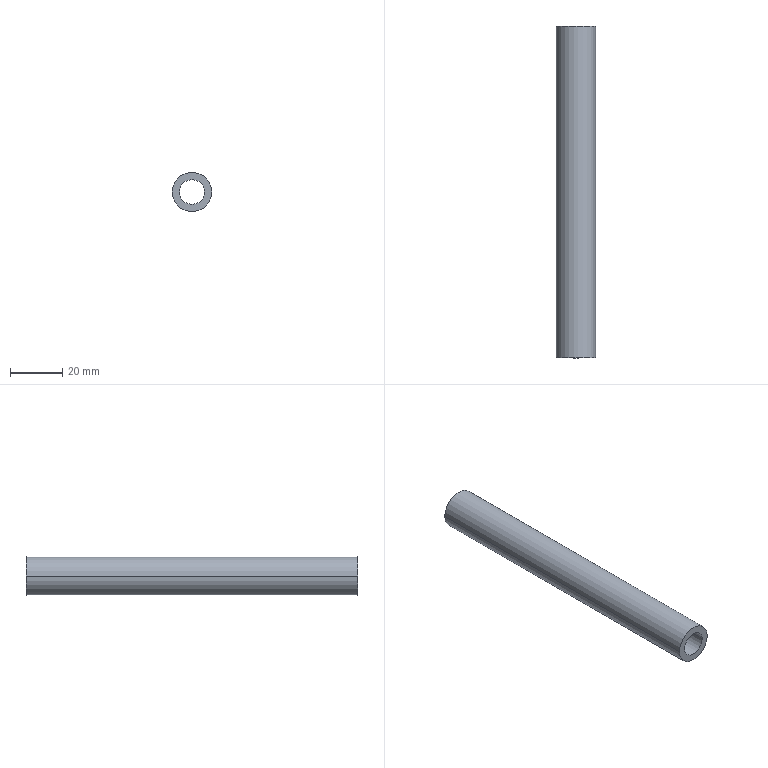Component | SolidWorks | MotorShaftHousing-2 | 1 solid | 6 faces | box 15 x 126.75 x 15 mm | volume 13414 mm3 | cylinder 4 | plane 2 | commonest cylinder face diameters 9.5 x2 15 x2
build123d program:
from build123d import *

# Parameters (mm, degrees)
BOSS_EXTRUDE1_DEPTH      = 51.75
BOSS_EXTRUDE1_DEPTH_BACK = 75
SKETCH1_R                = 7.5
SKETCH1_R_2              = 4.75


with BuildPart() as part:
    # Sketch1 → Boss-Extrude1 (new, two sides: drawn at the far end of the back side and taken through both)
    with BuildSketch(Plane.XY.offset(-BOSS_EXTRUDE1_DEPTH_BACK)):
        with Locations((255, -40)):
            Circle(SKETCH1_R)
        with Locations((255, -40)):
            Circle(SKETCH1_R_2, mode=Mode.SUBTRACT)
    extrude(amount=BOSS_EXTRUDE1_DEPTH + BOSS_EXTRUDE1_DEPTH_BACK)


solid = part.part

# Placed as in the assembly
solid = solid.moved(Location((10, 246.75, 70), (90, 0, 0)))
STEP:
#1=COLOUR_RGB('',0.7922,0.8196,0.9333);
#2=FILL_AREA_STYLE_COLOUR('',#1);
#3=FILL_AREA_STYLE('',(#2));
#4=SURFACE_STYLE_FILL_AREA(#3);
#5=SURFACE_SIDE_STYLE('',(#4));
#6=SURFACE_STYLE_USAGE(.BOTH.,#5);
#7=PRESENTATION_STYLE_ASSIGNMENT((#6));
#8=CARTESIAN_POINT('',(10.62,7.677,1.181));
#9=VERTEX_POINT('',#8);
#10=CARTESIAN_POINT('',(10.246,7.677,1.181));
#11=VERTEX_POINT('',#10);
#12=CARTESIAN_POINT('',(10.433,7.677,1.181));
#13=DIRECTION('',(0.,-1.,0.));
#14=DIRECTION('',(1.,0.,0.));
#15=AXIS2_PLACEMENT_3D('',#12,#13,#14);
#16=CIRCLE('',#15,0.187);
#17=EDGE_CURVE('',#9,#11,#16,.T.);
#18=ORIENTED_EDGE('',*,*,#17,.T.);
#19=CARTESIAN_POINT('',(10.246,12.667,1.181));
#20=VERTEX_POINT('',#19);
#21=CARTESIAN_POINT('',(10.246,6.842,1.181));
#22=DIRECTION('',(0.,1.,0.));
#23=VECTOR('',#22,39.37);
#24=LINE('',#21,#23);
#25=EDGE_CURVE('',#11,#20,#24,.T.);
#26=ORIENTED_EDGE('',*,*,#25,.T.);
#27=CARTESIAN_POINT('',(10.62,12.667,1.181));
#28=VERTEX_POINT('',#27);
#29=CARTESIAN_POINT('',(10.433,12.667,1.181));
#30=DIRECTION('',(-0.,1.,0.));
#31=DIRECTION('',(1.,0.,0.));
#32=AXIS2_PLACEMENT_3D('',#29,#30,#31);
#33=CIRCLE('',#32,0.187);
#34=EDGE_CURVE('',#20,#28,#33,.T.);
#35=ORIENTED_EDGE('',*,*,#34,.T.);
#36=CARTESIAN_POINT('',(10.62,6.842,1.181));
#37=DIRECTION('',(0.,1.,0.));
#38=VECTOR('',#37,39.37);
#39=LINE('',#36,#38);
#40=EDGE_CURVE('',#9,#28,#39,.T.);
#41=ORIENTED_EDGE('',*,*,#40,.F.);
#42=EDGE_LOOP('',(#18,#26,#35,#41));
#43=FACE_OUTER_BOUND('',#42,.T.);
#44=CARTESIAN_POINT('',(10.433,6.842,1.181));
#45=DIRECTION('',(0.,1.,0.));
#46=DIRECTION('',(1.,0.,0.));
#47=AXIS2_PLACEMENT_3D('',#44,#45,#46);
#48=CYLINDRICAL_SURFACE('',#47,0.187);
#49=ADVANCED_FACE('',(#43),#48,.F.);
#50=CARTESIAN_POINT('',(10.138,7.677,1.181));
#51=VERTEX_POINT('',#50);
#52=CARTESIAN_POINT('',(10.728,7.677,1.181));
#53=VERTEX_POINT('',#52);
#54=CARTESIAN_POINT('',(10.433,7.677,1.181));
#55=DIRECTION('',(0.,-1.,0.));
#56=DIRECTION('',(1.,0.,0.));
#57=AXIS2_PLACEMENT_3D('',#54,#55,#56);
#58=CIRCLE('',#57,0.2953);
#59=EDGE_CURVE('',#51,#53,#58,.T.);
#60=ORIENTED_EDGE('',*,*,#59,.F.);
#61=CARTESIAN_POINT('',(10.138,12.667,1.181));
#62=VERTEX_POINT('',#61);
#63=CARTESIAN_POINT('',(10.138,6.842,1.181));
#64=DIRECTION('',(0.,1.,0.));
#65=VECTOR('',#64,39.37);
#66=LINE('',#63,#65);
#67=EDGE_CURVE('',#51,#62,#66,.T.);
#68=ORIENTED_EDGE('',*,*,#67,.T.);
#69=CARTESIAN_POINT('',(10.728,12.667,1.181));
#70=VERTEX_POINT('',#69);
#71=CARTESIAN_POINT('',(10.433,12.667,1.181));
#72=DIRECTION('',(-0.,1.,0.));
#73=DIRECTION('',(1.,0.,0.));
#74=AXIS2_PLACEMENT_3D('',#71,#72,#73);
#75=CIRCLE('',#74,0.2953);
#76=EDGE_CURVE('',#70,#62,#75,.T.);
#77=ORIENTED_EDGE('',*,*,#76,.F.);
#78=CARTESIAN_POINT('',(10.728,6.842,1.181));
#79=DIRECTION('',(0.,1.,0.));
#80=VECTOR('',#79,39.37);
#81=LINE('',#78,#80);
#82=EDGE_CURVE('',#53,#70,#81,.T.);
#83=ORIENTED_EDGE('',*,*,#82,.F.);
#84=EDGE_LOOP('',(#60,#68,#77,#83));
#85=FACE_OUTER_BOUND('',#84,.T.);
#86=CARTESIAN_POINT('',(10.433,6.842,1.181));
#87=DIRECTION('',(0.,1.,0.));
#88=DIRECTION('',(1.,0.,0.));
#89=AXIS2_PLACEMENT_3D('',#86,#87,#88);
#90=CYLINDRICAL_SURFACE('',#89,0.2953);
#91=ADVANCED_FACE('',(#85),#90,.T.);
#92=ORIENTED_EDGE('',*,*,#67,.F.);
#93=CARTESIAN_POINT('',(10.433,7.677,1.181));
#94=DIRECTION('',(0.,-1.,0.));
#95=DIRECTION('',(1.,0.,0.));
#96=AXIS2_PLACEMENT_3D('',#93,#94,#95);
#97=CIRCLE('',#96,0.2953);
#98=EDGE_CURVE('',#53,#51,#97,.T.);
#99=ORIENTED_EDGE('',*,*,#98,.F.);
#100=ORIENTED_EDGE('',*,*,#82,.T.);
#101=CARTESIAN_POINT('',(10.433,12.667,1.181));
#102=DIRECTION('',(-0.,1.,0.));
#103=DIRECTION('',(1.,0.,0.));
#104=AXIS2_PLACEMENT_3D('',#101,#102,#103);
#105=CIRCLE('',#104,0.2953);
#106=EDGE_CURVE('',#62,#70,#105,.T.);
#107=ORIENTED_EDGE('',*,*,#106,.F.);
#108=EDGE_LOOP('',(#92,#99,#100,#107));
#109=FACE_OUTER_BOUND('',#108,.T.);
#110=CARTESIAN_POINT('',(10.433,6.842,1.181));
#111=DIRECTION('',(0.,1.,0.));
#112=DIRECTION('',(1.,0.,0.));
#113=AXIS2_PLACEMENT_3D('',#110,#111,#112);
#114=CYLINDRICAL_SURFACE('',#113,0.2953);
#115=ADVANCED_FACE('',(#109),#114,.T.);
#116=ORIENTED_EDGE('',*,*,#25,.F.);
#117=CARTESIAN_POINT('',(10.433,7.677,1.181));
#118=DIRECTION('',(0.,-1.,0.));
#119=DIRECTION('',(1.,0.,0.));
#120=AXIS2_PLACEMENT_3D('',#117,#118,#119);
#121=CIRCLE('',#120,0.187);
#122=EDGE_CURVE('',#11,#9,#121,.T.);
#123=ORIENTED_EDGE('',*,*,#122,.T.);
#124=ORIENTED_EDGE('',*,*,#40,.T.);
#125=CARTESIAN_POINT('',(10.433,12.667,1.181));
#126=DIRECTION('',(-0.,1.,0.));
#127=DIRECTION('',(1.,0.,0.));
#128=AXIS2_PLACEMENT_3D('',#125,#126,#127);
#129=CIRCLE('',#128,0.187);
#130=EDGE_CURVE('',#28,#20,#129,.T.);
#131=ORIENTED_EDGE('',*,*,#130,.T.);
#132=EDGE_LOOP('',(#116,#123,#124,#131));
#133=FACE_OUTER_BOUND('',#132,.T.);
#134=CARTESIAN_POINT('',(10.433,6.842,1.181));
#135=DIRECTION('',(0.,1.,0.));
#136=DIRECTION('',(1.,0.,0.));
#137=AXIS2_PLACEMENT_3D('',#134,#135,#136);
#138=CYLINDRICAL_SURFACE('',#137,0.187);
#139=ADVANCED_FACE('',(#133),#138,.F.);
#140=ORIENTED_EDGE('',*,*,#98,.T.);
#141=ORIENTED_EDGE('',*,*,#59,.T.);
#142=EDGE_LOOP('',(#140,#141));
#143=FACE_OUTER_BOUND('',#142,.T.);
#144=ORIENTED_EDGE('',*,*,#17,.F.);
#145=ORIENTED_EDGE('',*,*,#122,.F.);
#146=EDGE_LOOP('',(#144,#145));
#147=FACE_BOUND('',#146,.T.);
#148=CARTESIAN_POINT('',(20.798,7.677,-0.3614));
#149=DIRECTION('',(0.,1.,0.));
#150=DIRECTION('',(1.,0.,0.));
#151=AXIS2_PLACEMENT_3D('',#148,#149,#150);
#152=PLANE('',#151);
#153=ADVANCED_FACE('',(#143,#147),#152,.F.);
#154=ORIENTED_EDGE('',*,*,#130,.F.);
#155=ORIENTED_EDGE('',*,*,#34,.F.);
#156=EDGE_LOOP('',(#154,#155));
#157=FACE_BOUND('',#156,.T.);
#158=ORIENTED_EDGE('',*,*,#76,.T.);
#159=ORIENTED_EDGE('',*,*,#106,.T.);
#160=EDGE_LOOP('',(#158,#159));
#161=FACE_OUTER_BOUND('',#160,.T.);
#162=CARTESIAN_POINT('',(10.655,12.667,1.418));
#163=DIRECTION('',(-0.,1.,0.));
#164=DIRECTION('',(-0.7307,-0.,0.6827));
#165=AXIS2_PLACEMENT_3D('',#162,#163,#164);
#166=PLANE('',#165);
#167=ADVANCED_FACE('',(#157,#161),#166,.T.);
#168=CLOSED_SHELL('',(#49,#91,#115,#139,#153,#167));
#169=MANIFOLD_SOLID_BREP('',#168);
#170=STYLED_ITEM('',(#7),#169);
#171=(LENGTH_UNIT()NAMED_UNIT(*)SI_UNIT($,.METRE.));
#172=LENGTH_MEASURE_WITH_UNIT(LENGTH_MEASURE(0.0254),#171);
#173=DIMENSIONAL_EXPONENTS(1.,0.,0.,0.,0.,0.,0.);
#174=(CONVERSION_BASED_UNIT('',#172)LENGTH_UNIT()NAMED_UNIT(#173));
#175=UNCERTAINTY_MEASURE_WITH_UNIT(LENGTH_MEASURE(0.00001),#174,'','');
#176=(NAMED_UNIT(*)PLANE_ANGLE_UNIT()SI_UNIT($,.RADIAN.));
#177=(NAMED_UNIT(*)SI_UNIT($,.STERADIAN.)SOLID_ANGLE_UNIT());
#178=(GEOMETRIC_REPRESENTATION_CONTEXT(3)GLOBAL_UNCERTAINTY_ASSIGNED_CONTEXT((#175))GLOBAL_UNIT_ASSIGNED_CONTEXT((#174,#176,#177))REPRESENTATION_CONTEXT('',''));
#179=MECHANICAL_DESIGN_GEOMETRIC_PRESENTATION_REPRESENTATION('',(#170),#178);
#180=PRESENTATION_LAYER_ASSIGNMENT('','',(#170));
#181=CARTESIAN_POINT('',(0.,0.,0.));
#182=DIRECTION('',(0.,0.,1.));
#183=DIRECTION('',(1.,0.,0.));
#184=AXIS2_PLACEMENT_3D('',#181,#182,#183);
#185=(LENGTH_UNIT()NAMED_UNIT(*)SI_UNIT($,.METRE.));
#186=LENGTH_MEASURE_WITH_UNIT(LENGTH_MEASURE(0.0254),#185);
#187=DIMENSIONAL_EXPONENTS(1.,0.,0.,0.,0.,0.,0.);
#188=(CONVERSION_BASED_UNIT('',#186)LENGTH_UNIT()NAMED_UNIT(#187));
#189=UNCERTAINTY_MEASURE_WITH_UNIT(LENGTH_MEASURE(0.00001),#188,'','');
#190=(NAMED_UNIT(*)PLANE_ANGLE_UNIT()SI_UNIT($,.RADIAN.));
#191=(NAMED_UNIT(*)SI_UNIT($,.STERADIAN.)SOLID_ANGLE_UNIT());
#192=(GEOMETRIC_REPRESENTATION_CONTEXT(3)GLOBAL_UNCERTAINTY_ASSIGNED_CONTEXT((#189))GLOBAL_UNIT_ASSIGNED_CONTEXT((#188,#190,#191))REPRESENTATION_CONTEXT('',''));
#193=ADVANCED_BREP_SHAPE_REPRESENTATION('',(#169,#184),#192);